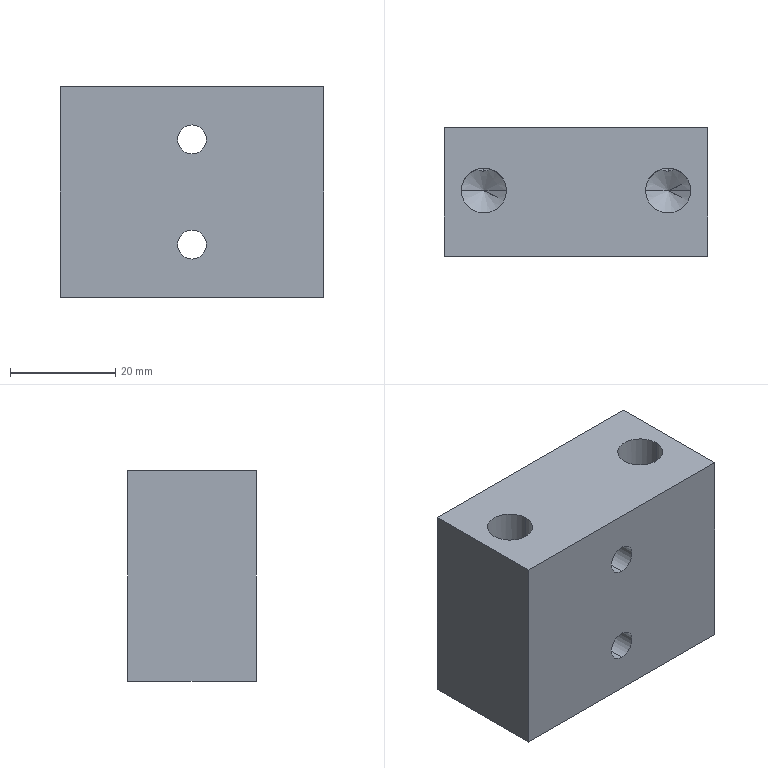Component | SolidWorks | F12529-M5107-1 | 1 solid | 32 faces | box 50 x 24.5 x 40 mm | volume 42311 mm3 | cylinder 20 | plane 8 | cone 4 | commonest cylinder face diameters 5 x8 10 x4 5.5 x4 8.566 x4 | material AISI 304
build123d program:
from build123d import *

# Parameters (mm, degrees)
SKETCH1_W                                            = 50
SKETCH1_H                                            = 40
EXTRUDE1_DEPTH                                       = 24.5
M5_TAPPED_HOLE1_D                                    = 5
M5_TAPPED_HOLE1_DEPTH                                = 12
M5_TAPPED_HOLE1_TIP                                  = 1.502
G1_8_THREADED_HOLE1_D                                = 8.566
G1_8_THREADED_HOLE1_DEPTH                            = 32.18
G1_8_THREADED_HOLE1_TIP                              = 2.573
M5_HEX_SOCKET_HEAD_CAP_SCREW_COUNTERBORE_D           = 5.5
M5_HEX_SOCKET_HEAD_CAP_SCREW_COUNTERBORE_CBORE_D     = 10
M5_HEX_SOCKET_HEAD_CAP_SCREW_COUNTERBORE_CBORE_DEPTH = 10


with BuildPart() as part:
    # Sketch1 → Extrude1 (new body)
    with BuildSketch(Plane(origin=(0, 0, 0), x_dir=(1, 0, 0), z_dir=(0, 1, 0))):
        Rectangle(SKETCH1_W, SKETCH1_H)
    extrude(amount=EXTRUDE1_DEPTH)

    # M5 Tapped Hole1
    with Locations(Plane(origin=(0, 24.5, 0), x_dir=(-1, 0, 0), z_dir=(0, 1, 0))):
        with Locations((17.5, -10), (17.5, 10), (-17.5, -10), (-17.5, 10)):
            Hole(M5_TAPPED_HOLE1_D / 2, depth=M5_TAPPED_HOLE1_DEPTH)
            with Locations((0, 0, -(M5_TAPPED_HOLE1_DEPTH + M5_TAPPED_HOLE1_TIP / 2))):  # 118° drill point
                Cone(0, M5_TAPPED_HOLE1_D / 2, M5_TAPPED_HOLE1_TIP, mode=Mode.SUBTRACT)

    # G1_8 Threaded Hole1
    with Locations(Plane.XY.offset(20)):
        with Locations((-17.5, 12.5), (17.5, 12.5)):
            Hole(G1_8_THREADED_HOLE1_D / 2, depth=G1_8_THREADED_HOLE1_DEPTH)
            with Locations((0, 0, -(G1_8_THREADED_HOLE1_DEPTH + G1_8_THREADED_HOLE1_TIP / 2))):  # 118° drill point
                Cone(0, G1_8_THREADED_HOLE1_D / 2, G1_8_THREADED_HOLE1_TIP, mode=Mode.SUBTRACT)

    # M5 Hex Socket Head Cap Screw Counterbore (through all)
    with Locations(Plane(origin=(0, 24.5, 0), x_dir=(-1, 0, 0), z_dir=(0, 1, 0))):
        with Locations((0, -10), (0, 10)):
            CounterBoreHole(M5_HEX_SOCKET_HEAD_CAP_SCREW_COUNTERBORE_D / 2, M5_HEX_SOCKET_HEAD_CAP_SCREW_COUNTERBORE_CBORE_D / 2, M5_HEX_SOCKET_HEAD_CAP_SCREW_COUNTERBORE_CBORE_DEPTH)


solid = part.part

# Placed as in the assembly
solid = solid.moved(Location((0, 203, 0), (0, 0, 0)))